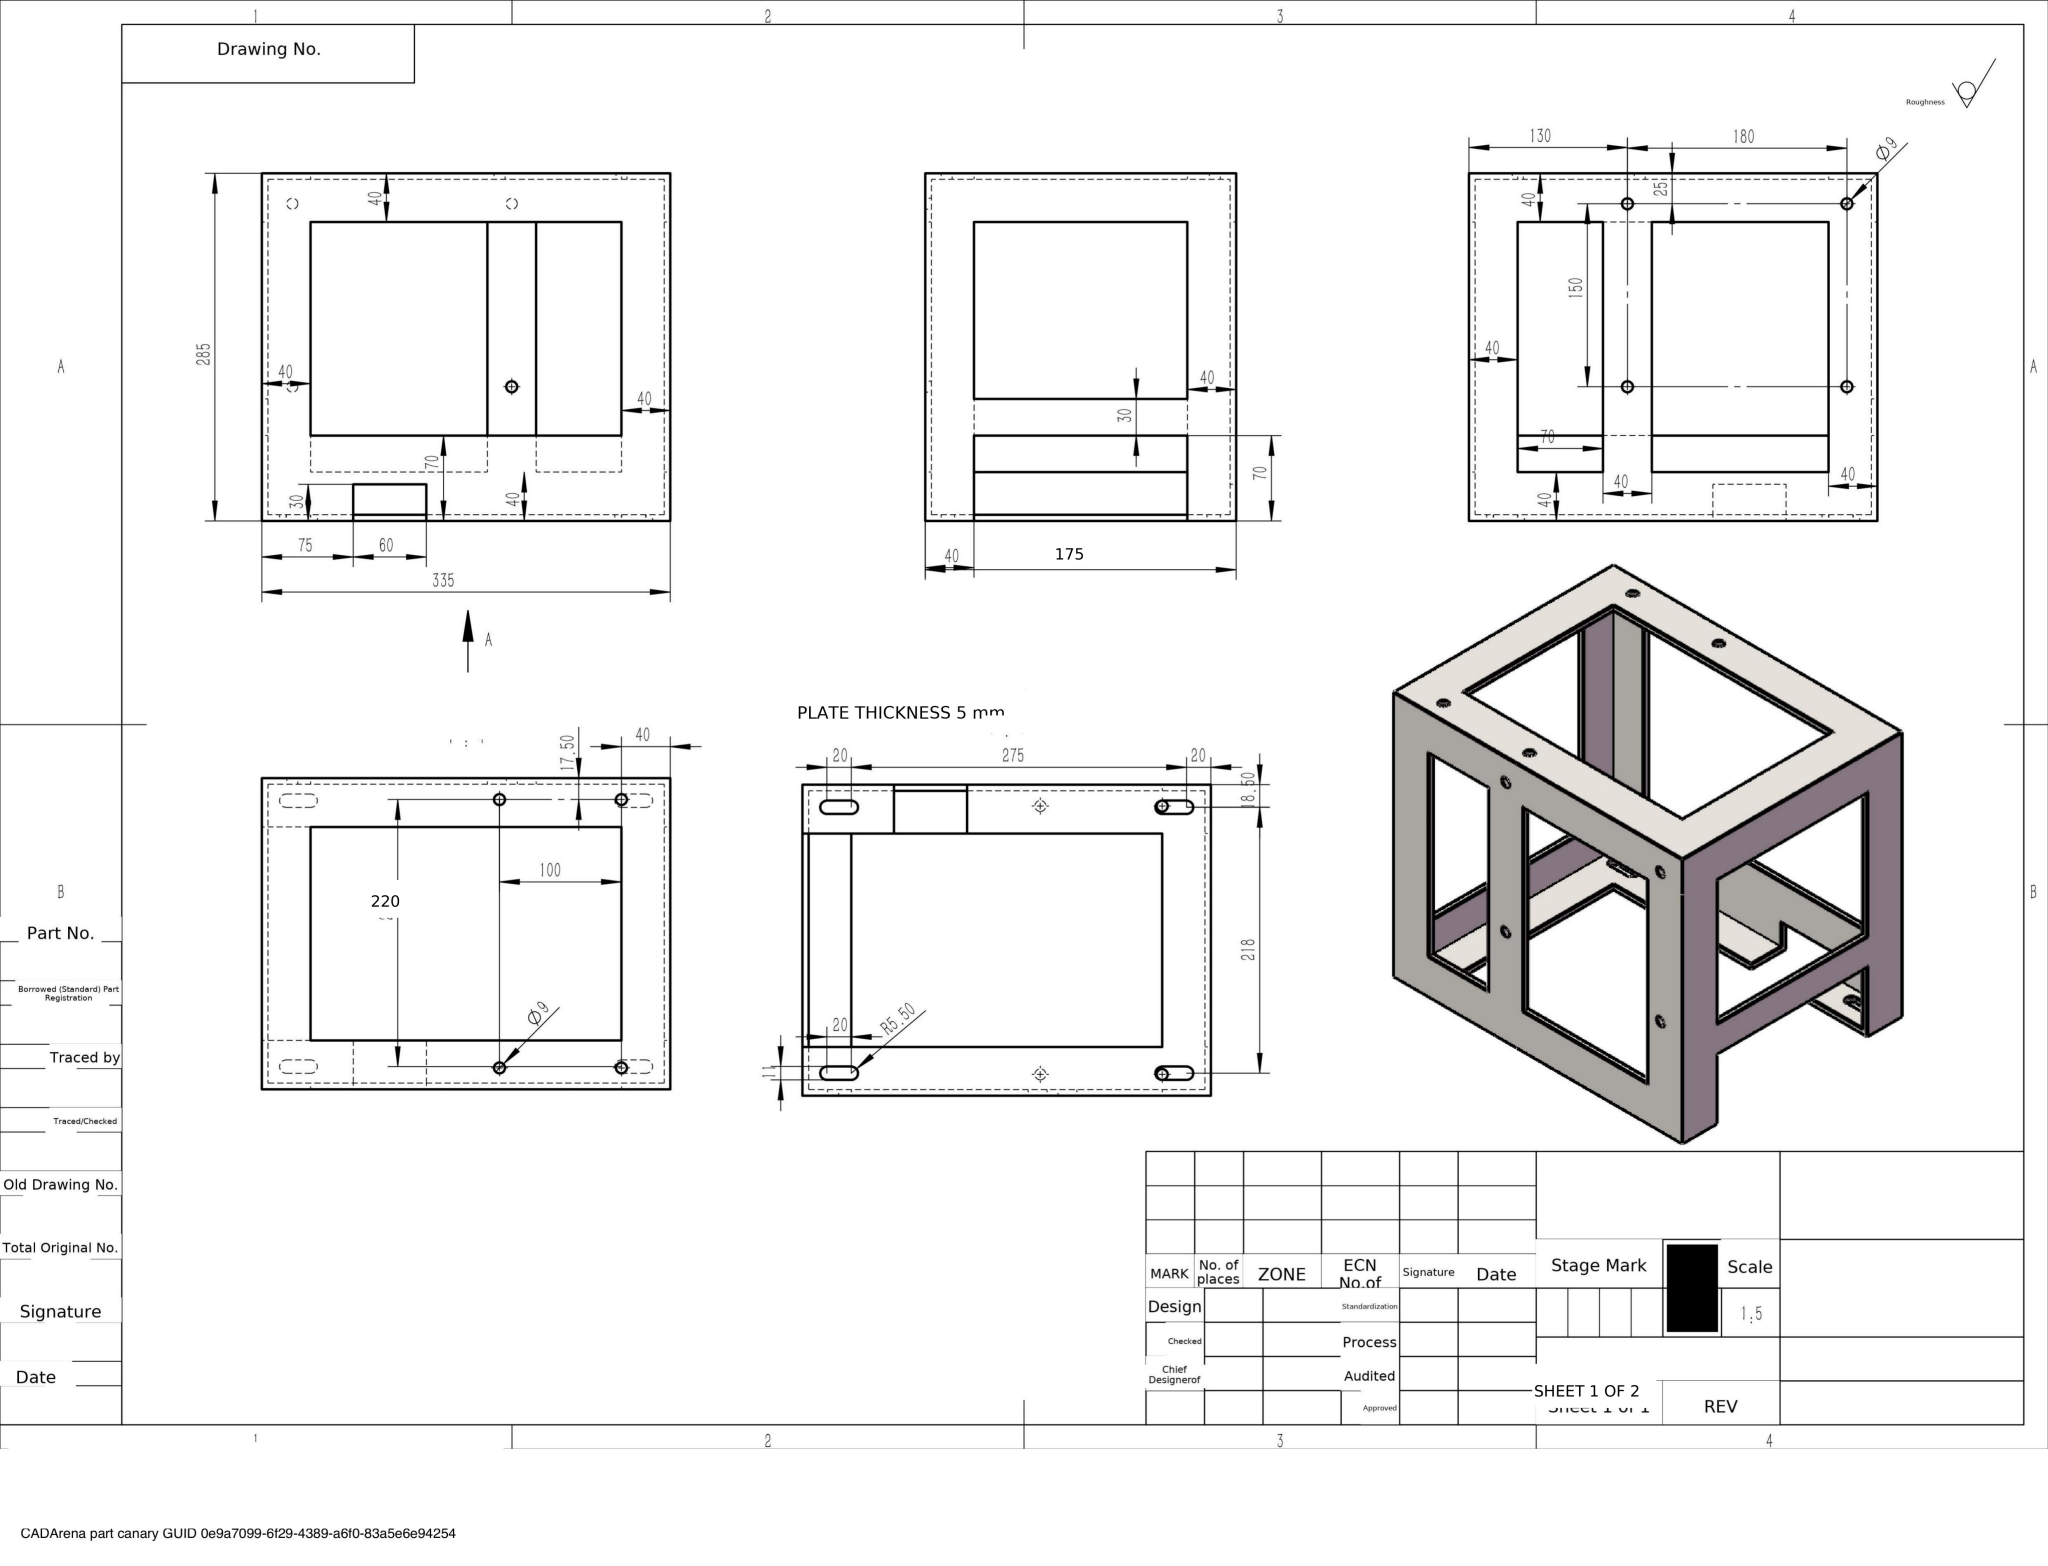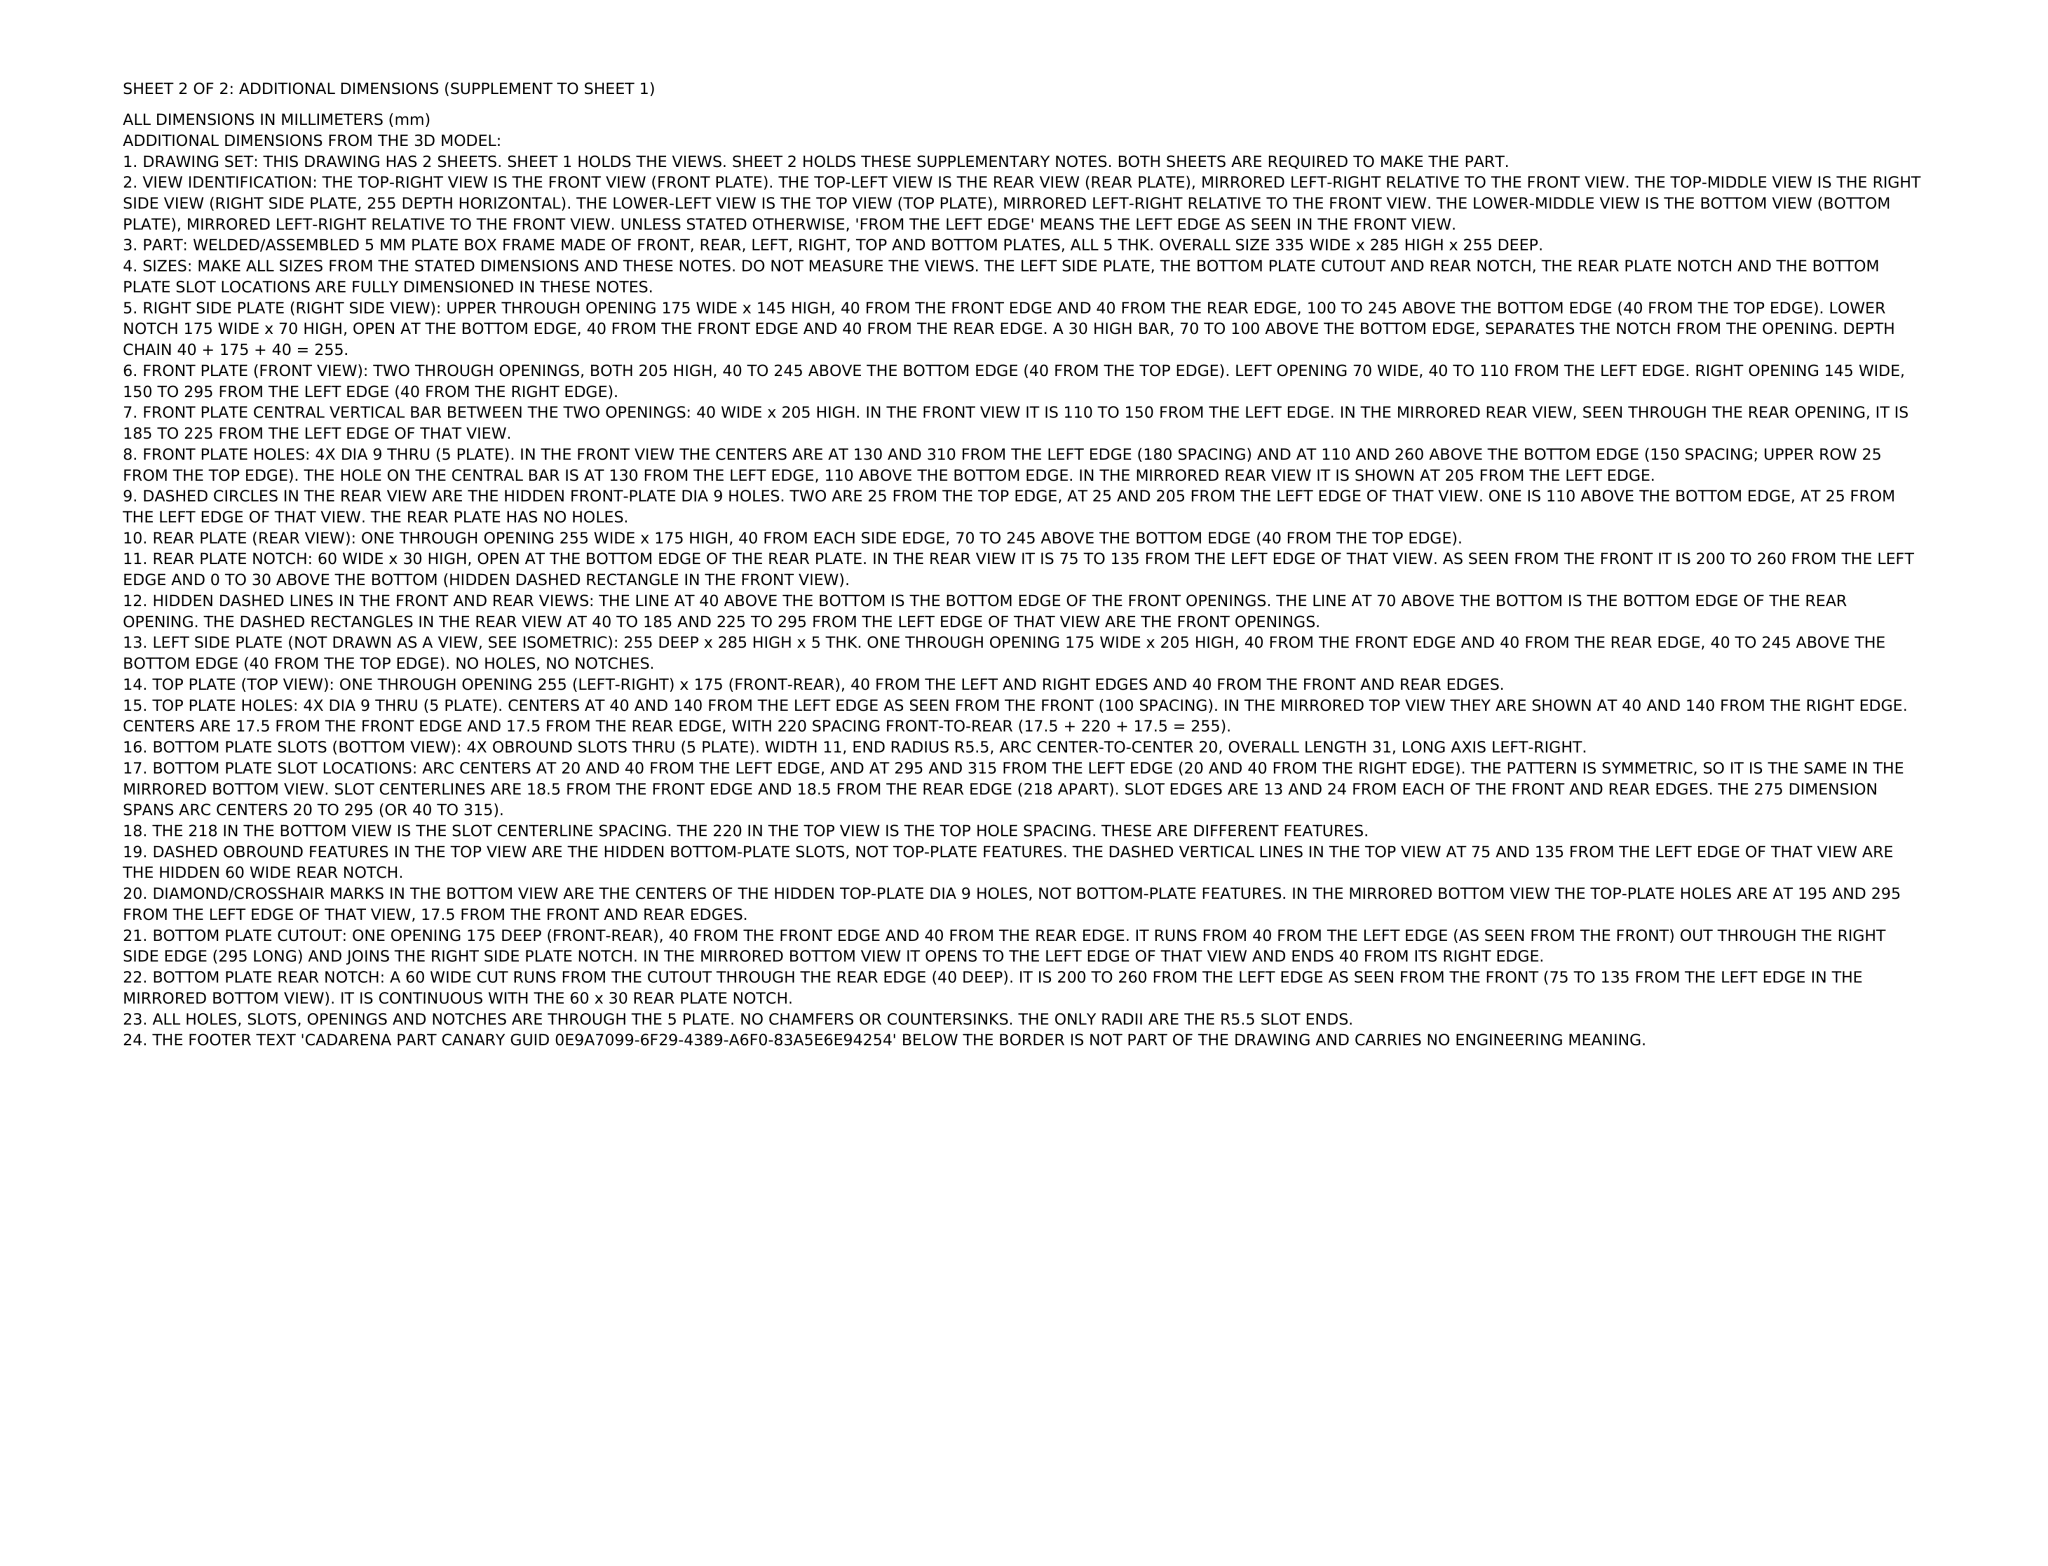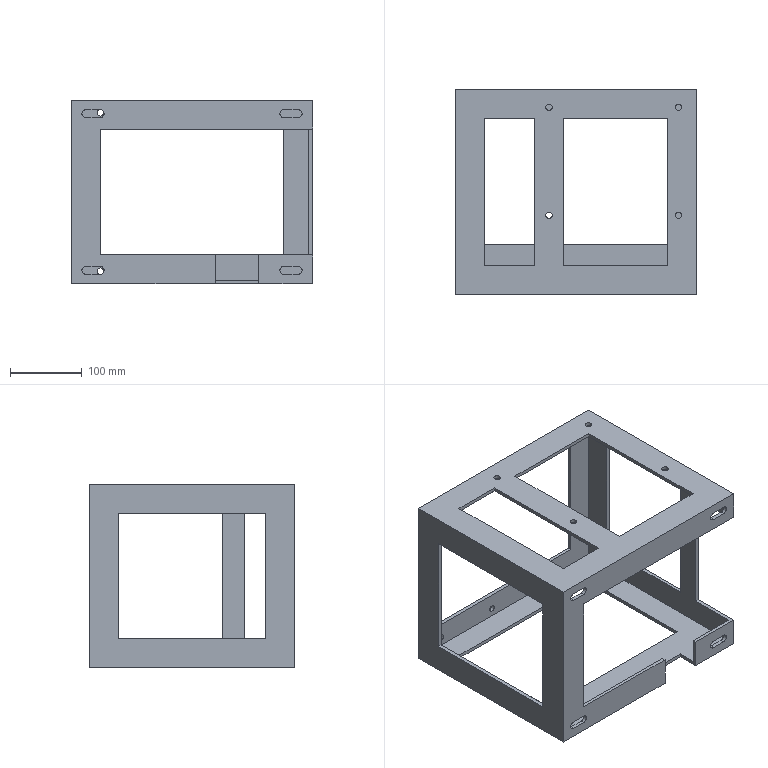Part | NX | mm | 1 solid | 78 faces | box 335 x 285 x 255 mm | volume 1133030 mm3 | plane 54 | cylinder 24 | commonest cylinder face diameters 9 x16 11 x8